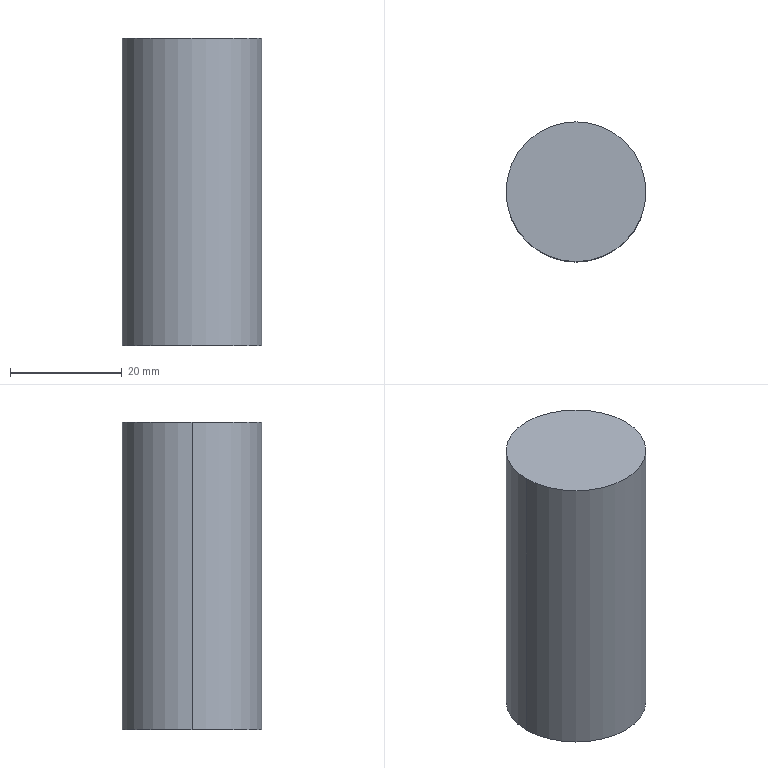Component | SolidWorks | Pin-1 | 1 solid | 4 faces | box 25 x 25 x 55 mm | volume 26998 mm3 | cylinder 2 | plane 2 | commonest cylinder face diameters 25 x2
build123d program:
from build123d import *

# Parameters (mm, degrees)
SKETCH1_R           = 12.5
BOSS_EXTRUDE1_DEPTH = 55


with BuildPart() as part:
    # Sketch1 → Boss-Extrude1 (new body)
    with BuildSketch(Plane.XY):
        Circle(SKETCH1_R)
    extrude(amount=BOSS_EXTRUDE1_DEPTH)


solid = part.part

# Placed as in the assembly
solid = solid.moved(Location((69.344, 1052.787, -10.5), (0, 0, 0)))
STEP:
#1=CARTESIAN_POINT('',(3.222,41.448,1.752));
#2=VERTEX_POINT('',#1);
#3=CARTESIAN_POINT('',(2.238,41.448,1.752));
#4=VERTEX_POINT('',#3);
#5=CARTESIAN_POINT('',(2.73,41.448,1.752));
#6=DIRECTION('',(0.,0.,1.));
#7=DIRECTION('',(1.,0.,0.));
#8=AXIS2_PLACEMENT_3D('',#5,#6,#7);
#9=CIRCLE('',#8,0.4921);
#10=EDGE_CURVE('',#2,#4,#9,.T.);
#11=ORIENTED_EDGE('',*,*,#10,.F.);
#12=CARTESIAN_POINT('',(3.222,41.448,-0.4134));
#13=VERTEX_POINT('',#12);
#14=CARTESIAN_POINT('',(3.222,41.448,1.752));
#15=DIRECTION('',(0.,0.,-1.));
#16=VECTOR('',#15,39.37);
#17=LINE('',#14,#16);
#18=EDGE_CURVE('',#2,#13,#17,.T.);
#19=ORIENTED_EDGE('',*,*,#18,.T.);
#20=CARTESIAN_POINT('',(2.238,41.448,-0.4134));
#21=VERTEX_POINT('',#20);
#22=CARTESIAN_POINT('',(2.73,41.448,-0.4134));
#23=DIRECTION('',(0.,0.,1.));
#24=DIRECTION('',(1.,0.,0.));
#25=AXIS2_PLACEMENT_3D('',#22,#23,#24);
#26=CIRCLE('',#25,0.4921);
#27=EDGE_CURVE('',#13,#21,#26,.T.);
#28=ORIENTED_EDGE('',*,*,#27,.T.);
#29=CARTESIAN_POINT('',(2.238,41.448,1.752));
#30=DIRECTION('',(0.,0.,-1.));
#31=VECTOR('',#30,39.37);
#32=LINE('',#29,#31);
#33=EDGE_CURVE('',#4,#21,#32,.T.);
#34=ORIENTED_EDGE('',*,*,#33,.F.);
#35=EDGE_LOOP('',(#11,#19,#28,#34));
#36=FACE_OUTER_BOUND('',#35,.T.);
#37=CARTESIAN_POINT('',(2.73,41.448,1.752));
#38=DIRECTION('',(0.,0.,-1.));
#39=DIRECTION('',(-1.,0.,0.));
#40=AXIS2_PLACEMENT_3D('',#37,#38,#39);
#41=CYLINDRICAL_SURFACE('',#40,0.4921);
#42=ADVANCED_FACE('',(#36),#41,.T.);
#43=ORIENTED_EDGE('',*,*,#18,.F.);
#44=CARTESIAN_POINT('',(2.73,41.448,1.752));
#45=DIRECTION('',(0.,0.,1.));
#46=DIRECTION('',(1.,0.,0.));
#47=AXIS2_PLACEMENT_3D('',#44,#45,#46);
#48=CIRCLE('',#47,0.4921);
#49=EDGE_CURVE('',#4,#2,#48,.T.);
#50=ORIENTED_EDGE('',*,*,#49,.F.);
#51=ORIENTED_EDGE('',*,*,#33,.T.);
#52=CARTESIAN_POINT('',(2.73,41.448,-0.4134));
#53=DIRECTION('',(0.,0.,1.));
#54=DIRECTION('',(1.,0.,0.));
#55=AXIS2_PLACEMENT_3D('',#52,#53,#54);
#56=CIRCLE('',#55,0.4921);
#57=EDGE_CURVE('',#21,#13,#56,.T.);
#58=ORIENTED_EDGE('',*,*,#57,.T.);
#59=EDGE_LOOP('',(#43,#50,#51,#58));
#60=FACE_OUTER_BOUND('',#59,.T.);
#61=CARTESIAN_POINT('',(2.73,41.448,1.752));
#62=DIRECTION('',(0.,0.,-1.));
#63=DIRECTION('',(-1.,0.,0.));
#64=AXIS2_PLACEMENT_3D('',#61,#62,#63);
#65=CYLINDRICAL_SURFACE('',#64,0.4921);
#66=ADVANCED_FACE('',(#60),#65,.T.);
#67=ORIENTED_EDGE('',*,*,#49,.T.);
#68=ORIENTED_EDGE('',*,*,#10,.T.);
#69=EDGE_LOOP('',(#67,#68));
#70=FACE_OUTER_BOUND('',#69,.T.);
#71=CARTESIAN_POINT('',(2.73,41.448,1.752));
#72=DIRECTION('',(0.,0.,1.));
#73=DIRECTION('',(1.,0.,0.));
#74=AXIS2_PLACEMENT_3D('',#71,#72,#73);
#75=PLANE('',#74);
#76=ADVANCED_FACE('',(#70),#75,.T.);
#77=ORIENTED_EDGE('',*,*,#57,.F.);
#78=ORIENTED_EDGE('',*,*,#27,.F.);
#79=EDGE_LOOP('',(#77,#78));
#80=FACE_OUTER_BOUND('',#79,.T.);
#81=CARTESIAN_POINT('',(2.73,41.448,-0.4134));
#82=DIRECTION('',(0.,0.,1.));
#83=DIRECTION('',(1.,0.,0.));
#84=AXIS2_PLACEMENT_3D('',#81,#82,#83);
#85=PLANE('',#84);
#86=ADVANCED_FACE('',(#80),#85,.F.);
#87=CLOSED_SHELL('',(#42,#66,#76,#86));
#88=MANIFOLD_SOLID_BREP('',#87);
#89=CARTESIAN_POINT('',(0.,0.,0.));
#90=DIRECTION('',(0.,0.,1.));
#91=DIRECTION('',(1.,0.,0.));
#92=AXIS2_PLACEMENT_3D('',#89,#90,#91);
#93=(LENGTH_UNIT()NAMED_UNIT(*)SI_UNIT($,.METRE.));
#94=LENGTH_MEASURE_WITH_UNIT(LENGTH_MEASURE(0.0254),#93);
#95=DIMENSIONAL_EXPONENTS(1.,0.,0.,0.,0.,0.,0.);
#96=(CONVERSION_BASED_UNIT('',#94)LENGTH_UNIT()NAMED_UNIT(#95));
#97=UNCERTAINTY_MEASURE_WITH_UNIT(LENGTH_MEASURE(0.00001),#96,'','');
#98=(NAMED_UNIT(*)PLANE_ANGLE_UNIT()SI_UNIT($,.RADIAN.));
#99=(NAMED_UNIT(*)SI_UNIT($,.STERADIAN.)SOLID_ANGLE_UNIT());
#100=(GEOMETRIC_REPRESENTATION_CONTEXT(3)GLOBAL_UNCERTAINTY_ASSIGNED_CONTEXT((#97))GLOBAL_UNIT_ASSIGNED_CONTEXT((#96,#98,#99))REPRESENTATION_CONTEXT('',''));
#101=ADVANCED_BREP_SHAPE_REPRESENTATION('',(#88,#92),#100);
#102=COLOUR_RGB('',0.7922,0.8196,0.9333);
#103=FILL_AREA_STYLE_COLOUR('',#102);
#104=FILL_AREA_STYLE('',(#103));
#105=SURFACE_STYLE_FILL_AREA(#104);
#106=SURFACE_SIDE_STYLE('',(#105));
#107=SURFACE_STYLE_USAGE(.BOTH.,#106);
#108=PRESENTATION_STYLE_ASSIGNMENT((#107));
#109=STYLED_ITEM('',(#108),#88);
#110=(LENGTH_UNIT()NAMED_UNIT(*)SI_UNIT($,.METRE.));
#111=LENGTH_MEASURE_WITH_UNIT(LENGTH_MEASURE(0.0254),#110);
#112=DIMENSIONAL_EXPONENTS(1.,0.,0.,0.,0.,0.,0.);
#113=(CONVERSION_BASED_UNIT('',#111)LENGTH_UNIT()NAMED_UNIT(#112));
#114=UNCERTAINTY_MEASURE_WITH_UNIT(LENGTH_MEASURE(0.00001),#113,'','');
#115=(NAMED_UNIT(*)PLANE_ANGLE_UNIT()SI_UNIT($,.RADIAN.));
#116=(NAMED_UNIT(*)SI_UNIT($,.STERADIAN.)SOLID_ANGLE_UNIT());
#117=(GEOMETRIC_REPRESENTATION_CONTEXT(3)GLOBAL_UNCERTAINTY_ASSIGNED_CONTEXT((#114))GLOBAL_UNIT_ASSIGNED_CONTEXT((#113,#115,#116))REPRESENTATION_CONTEXT('',''));
#118=MECHANICAL_DESIGN_GEOMETRIC_PRESENTATION_REPRESENTATION('',(#109),#117);
#119=PRESENTATION_LAYER_ASSIGNMENT('','',(#109));